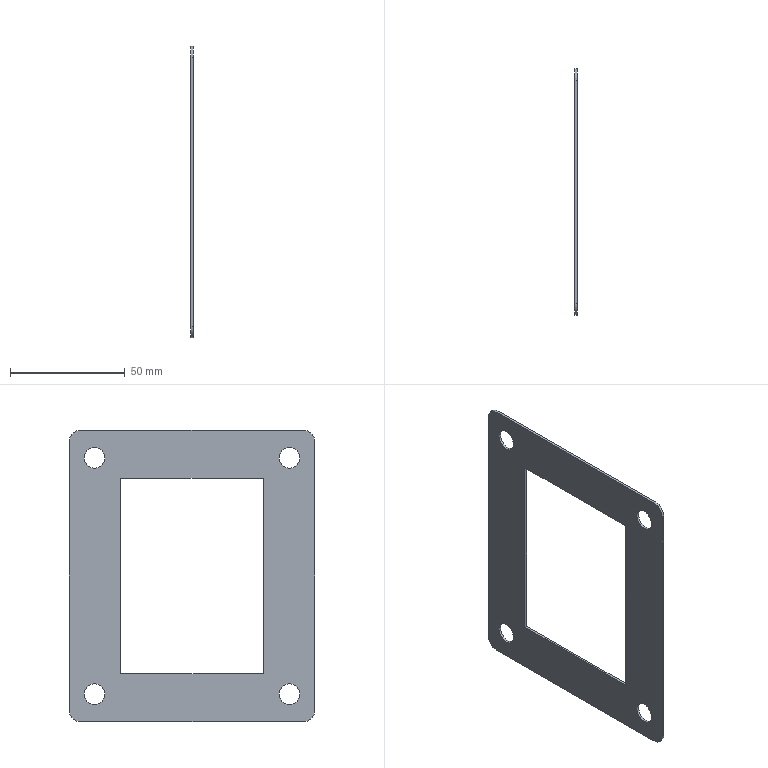Component | SolidWorks | 17-1 | 1 solid | 22 faces | box 1 x 107 x 127 mm | volume 8043 mm3 | cylinder 12 | plane 10 | commonest cylinder face diameters 9 x8 10 x4
build123d program:
from build123d import *

# Parameters (mm, degrees)
SKETCH1_R           = 4.5
SKETCH1_W           = 85
SKETCH1_H           = 62
BOSS_EXTRUDE1_DEPTH = 1


with BuildPart() as part:
    # Sketch1 → Boss-Extrude1 (new body)
    with BuildSketch(Plane(origin=(0, 0, 0), x_dir=(1, 0, 0), z_dir=(0, 1, 0))):
        with BuildLine():
            Line((-58.5, -53.5), (58.5, -53.5))
            ThreePointArc((58.5, -53.5), (62.036, -52.036), (63.5, -48.5))
            Line((63.5, -48.5), (63.5, 48.5))
            ThreePointArc((63.5, 48.5), (62.036, 52.036), (58.5, 53.5))
            Line((58.5, 53.5), (-58.5, 53.5))
            ThreePointArc((-58.5, 53.5), (-62.036, 52.036), (-63.5, 48.5))
            Line((-63.5, 48.5), (-63.5, -48.5))
            ThreePointArc((-63.5, -48.5), (-62.036, -52.036), (-58.5, -53.5))
        make_face()
        with Locations(Location((-51.5, 42.5, 0), (0, 0, 270))):
            Circle(SKETCH1_R, mode=Mode.SUBTRACT)
        with Locations(Location((51.5, 42.5, 0), (0, 0, 270))):
            Circle(SKETCH1_R, mode=Mode.SUBTRACT)
        with Locations(Location((51.5, -42.5, 0), (0, 0, 90))):
            Circle(SKETCH1_R, mode=Mode.SUBTRACT)
        with Locations(Location((-51.5, -42.5, 0), (0, 0, 90))):
            Circle(SKETCH1_R, mode=Mode.SUBTRACT)
        Rectangle(SKETCH1_W, SKETCH1_H, mode=Mode.SUBTRACT)
    extrude(amount=BOSS_EXTRUDE1_DEPTH)


solid = part.part

# Placed as in the assembly
solid = solid.moved(Location((-85, -47, 0), (90, 0, 90)))